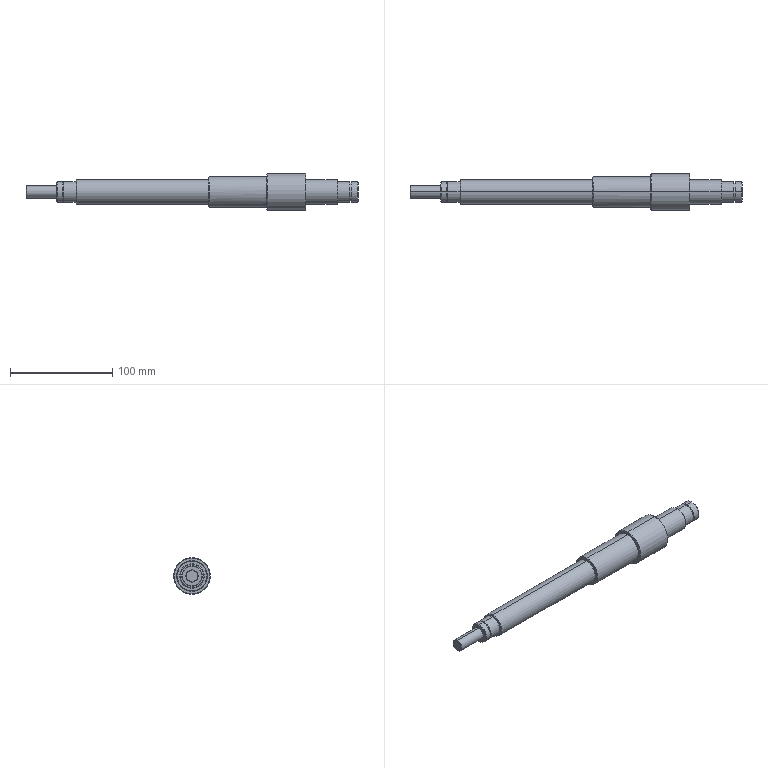CAM job | Mastercam | mm | 1 operations | part box 355 x 36 x 36
1. Contour (Ramp) | 3 - 3 平铣刀